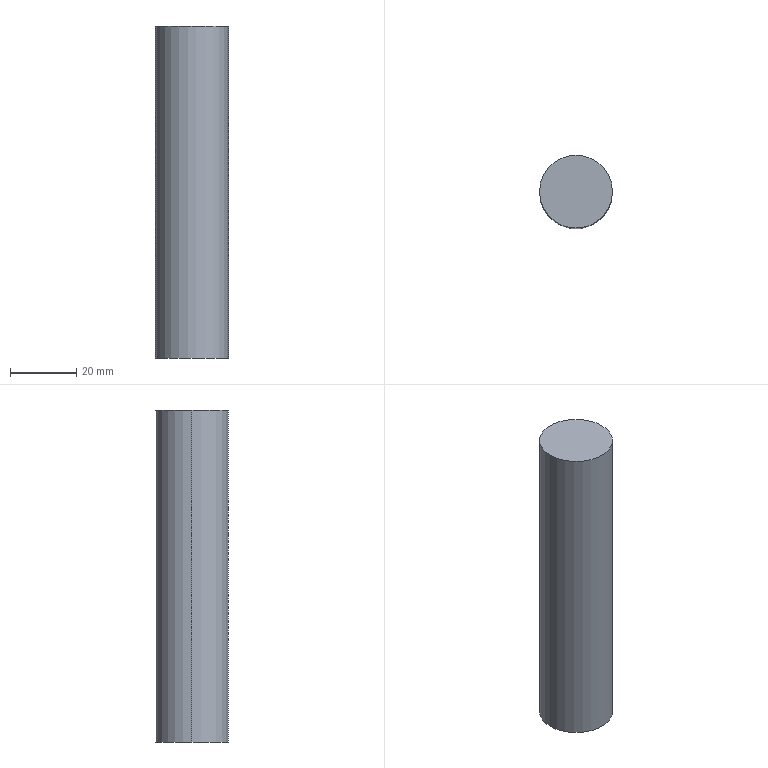Component | SolidWorks | AD12-daozhu.SDPRT-1 | 1 solid | 4 faces | box 22 x 22 x 100 mm | volume 38013 mm3 | cylinder 2 | plane 2 | commonest cylinder face diameters 22 x2
build123d program:
from build123d import *

# Parameters (mm, degrees)
SKETCH1_R           = 11
BOSS_EXTRUDE1_DEPTH = 100


with BuildPart() as part:
    # Sketch1 → Boss-Extrude1 (new body)
    with BuildSketch(Plane.XY):
        Circle(SKETCH1_R)
    extrude(amount=BOSS_EXTRUDE1_DEPTH)


solid = part.part

# Placed as in the assembly
solid = solid.moved(Location((-359.414, 119.039, 244.12), (0, 0, 0)))
STEP:
#1=COLOUR_RGB('',0.7922,0.8196,0.9333);
#2=FILL_AREA_STYLE_COLOUR('',#1);
#3=FILL_AREA_STYLE('',(#2));
#4=SURFACE_STYLE_FILL_AREA(#3);
#5=SURFACE_SIDE_STYLE('',(#4));
#6=SURFACE_STYLE_USAGE(.BOTH.,#5);
#7=PRESENTATION_STYLE_ASSIGNMENT((#6));
#8=CARTESIAN_POINT('',(-13.717,4.687,13.548));
#9=VERTEX_POINT('',#8);
#10=CARTESIAN_POINT('',(-14.583,4.687,13.548));
#11=VERTEX_POINT('',#10);
#12=CARTESIAN_POINT('',(-14.15,4.687,13.548));
#13=DIRECTION('',(0.,0.,1.));
#14=DIRECTION('',(1.,0.,0.));
#15=AXIS2_PLACEMENT_3D('',#12,#13,#14);
#16=CIRCLE('',#15,0.4331);
#17=EDGE_CURVE('',#9,#11,#16,.T.);
#18=ORIENTED_EDGE('',*,*,#17,.F.);
#19=CARTESIAN_POINT('',(-13.717,4.687,9.611));
#20=VERTEX_POINT('',#19);
#21=CARTESIAN_POINT('',(-13.717,4.687,13.548));
#22=DIRECTION('',(0.,0.,-1.));
#23=VECTOR('',#22,39.37);
#24=LINE('',#21,#23);
#25=EDGE_CURVE('',#9,#20,#24,.T.);
#26=ORIENTED_EDGE('',*,*,#25,.T.);
#27=CARTESIAN_POINT('',(-14.583,4.687,9.611));
#28=VERTEX_POINT('',#27);
#29=CARTESIAN_POINT('',(-14.15,4.687,9.611));
#30=DIRECTION('',(0.,0.,1.));
#31=DIRECTION('',(1.,0.,0.));
#32=AXIS2_PLACEMENT_3D('',#29,#30,#31);
#33=CIRCLE('',#32,0.4331);
#34=EDGE_CURVE('',#20,#28,#33,.T.);
#35=ORIENTED_EDGE('',*,*,#34,.T.);
#36=CARTESIAN_POINT('',(-14.583,4.687,13.548));
#37=DIRECTION('',(0.,0.,-1.));
#38=VECTOR('',#37,39.37);
#39=LINE('',#36,#38);
#40=EDGE_CURVE('',#11,#28,#39,.T.);
#41=ORIENTED_EDGE('',*,*,#40,.F.);
#42=EDGE_LOOP('',(#18,#26,#35,#41));
#43=FACE_OUTER_BOUND('',#42,.T.);
#44=CARTESIAN_POINT('',(-14.15,4.687,13.548));
#45=DIRECTION('',(0.,0.,-1.));
#46=DIRECTION('',(-1.,0.,0.));
#47=AXIS2_PLACEMENT_3D('',#44,#45,#46);
#48=CYLINDRICAL_SURFACE('',#47,0.4331);
#49=ADVANCED_FACE('',(#43),#48,.T.);
#50=ORIENTED_EDGE('',*,*,#25,.F.);
#51=CARTESIAN_POINT('',(-14.15,4.687,13.548));
#52=DIRECTION('',(0.,0.,1.));
#53=DIRECTION('',(1.,0.,0.));
#54=AXIS2_PLACEMENT_3D('',#51,#52,#53);
#55=CIRCLE('',#54,0.4331);
#56=EDGE_CURVE('',#11,#9,#55,.T.);
#57=ORIENTED_EDGE('',*,*,#56,.F.);
#58=ORIENTED_EDGE('',*,*,#40,.T.);
#59=CARTESIAN_POINT('',(-14.15,4.687,9.611));
#60=DIRECTION('',(0.,0.,1.));
#61=DIRECTION('',(1.,0.,0.));
#62=AXIS2_PLACEMENT_3D('',#59,#60,#61);
#63=CIRCLE('',#62,0.4331);
#64=EDGE_CURVE('',#28,#20,#63,.T.);
#65=ORIENTED_EDGE('',*,*,#64,.T.);
#66=EDGE_LOOP('',(#50,#57,#58,#65));
#67=FACE_OUTER_BOUND('',#66,.T.);
#68=CARTESIAN_POINT('',(-14.15,4.687,13.548));
#69=DIRECTION('',(0.,0.,-1.));
#70=DIRECTION('',(-1.,0.,0.));
#71=AXIS2_PLACEMENT_3D('',#68,#69,#70);
#72=CYLINDRICAL_SURFACE('',#71,0.4331);
#73=ADVANCED_FACE('',(#67),#72,.T.);
#74=ORIENTED_EDGE('',*,*,#56,.T.);
#75=ORIENTED_EDGE('',*,*,#17,.T.);
#76=EDGE_LOOP('',(#74,#75));
#77=FACE_OUTER_BOUND('',#76,.T.);
#78=CARTESIAN_POINT('',(-14.15,4.687,13.548));
#79=DIRECTION('',(0.,0.,1.));
#80=DIRECTION('',(1.,0.,0.));
#81=AXIS2_PLACEMENT_3D('',#78,#79,#80);
#82=PLANE('',#81);
#83=ADVANCED_FACE('',(#77),#82,.T.);
#84=ORIENTED_EDGE('',*,*,#64,.F.);
#85=ORIENTED_EDGE('',*,*,#34,.F.);
#86=EDGE_LOOP('',(#84,#85));
#87=FACE_OUTER_BOUND('',#86,.T.);
#88=CARTESIAN_POINT('',(-14.15,4.687,9.611));
#89=DIRECTION('',(0.,0.,1.));
#90=DIRECTION('',(1.,0.,0.));
#91=AXIS2_PLACEMENT_3D('',#88,#89,#90);
#92=PLANE('',#91);
#93=ADVANCED_FACE('',(#87),#92,.F.);
#94=CLOSED_SHELL('',(#49,#73,#83,#93));
#95=MANIFOLD_SOLID_BREP('',#94);
#96=STYLED_ITEM('',(#7),#95);
#97=PRESENTATION_LAYER_ASSIGNMENT('','',(#96));
#98=(LENGTH_UNIT()NAMED_UNIT(*)SI_UNIT($,.METRE.));
#99=LENGTH_MEASURE_WITH_UNIT(LENGTH_MEASURE(0.0254),#98);
#100=DIMENSIONAL_EXPONENTS(1.,0.,0.,0.,0.,0.,0.);
#101=(CONVERSION_BASED_UNIT('',#99)LENGTH_UNIT()NAMED_UNIT(#100));
#102=UNCERTAINTY_MEASURE_WITH_UNIT(LENGTH_MEASURE(0.00001),#101,'','');
#103=(NAMED_UNIT(*)PLANE_ANGLE_UNIT()SI_UNIT($,.RADIAN.));
#104=(NAMED_UNIT(*)SI_UNIT($,.STERADIAN.)SOLID_ANGLE_UNIT());
#105=(GEOMETRIC_REPRESENTATION_CONTEXT(3)GLOBAL_UNCERTAINTY_ASSIGNED_CONTEXT((#102))GLOBAL_UNIT_ASSIGNED_CONTEXT((#101,#103,#104))REPRESENTATION_CONTEXT('',''));
#106=MECHANICAL_DESIGN_GEOMETRIC_PRESENTATION_REPRESENTATION('',(#96),#105);
#107=CARTESIAN_POINT('',(0.,0.,0.));
#108=DIRECTION('',(0.,0.,1.));
#109=DIRECTION('',(1.,0.,0.));
#110=AXIS2_PLACEMENT_3D('',#107,#108,#109);
#111=(LENGTH_UNIT()NAMED_UNIT(*)SI_UNIT($,.METRE.));
#112=LENGTH_MEASURE_WITH_UNIT(LENGTH_MEASURE(0.0254),#111);
#113=DIMENSIONAL_EXPONENTS(1.,0.,0.,0.,0.,0.,0.);
#114=(CONVERSION_BASED_UNIT('',#112)LENGTH_UNIT()NAMED_UNIT(#113));
#115=UNCERTAINTY_MEASURE_WITH_UNIT(LENGTH_MEASURE(0.00001),#114,'','');
#116=(NAMED_UNIT(*)PLANE_ANGLE_UNIT()SI_UNIT($,.RADIAN.));
#117=(NAMED_UNIT(*)SI_UNIT($,.STERADIAN.)SOLID_ANGLE_UNIT());
#118=(GEOMETRIC_REPRESENTATION_CONTEXT(3)GLOBAL_UNCERTAINTY_ASSIGNED_CONTEXT((#115))GLOBAL_UNIT_ASSIGNED_CONTEXT((#114,#116,#117))REPRESENTATION_CONTEXT('',''));
#119=ADVANCED_BREP_SHAPE_REPRESENTATION('',(#95,#110),#118);